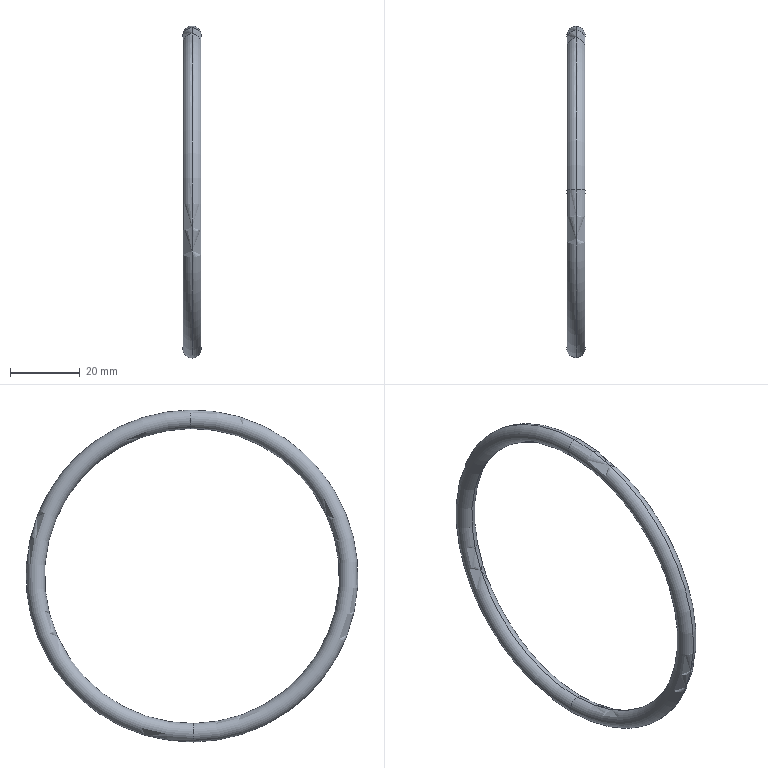Component | SolidWorks | SpringClipRubberRing-1 | 1 solid | 4 faces | box 5.3 x 95.03 x 95.03 mm | volume 6219 mm3 | torus 4 | material Silicone Rubber
STEP:
#1=COLOUR_RGB('',0.7922,0.8196,0.9333);
#2=FILL_AREA_STYLE_COLOUR('',#1);
#3=FILL_AREA_STYLE('',(#2));
#4=SURFACE_STYLE_FILL_AREA(#3);
#5=SURFACE_SIDE_STYLE('',(#4));
#6=SURFACE_STYLE_USAGE(.BOTH.,#5);
#7=PRESENTATION_STYLE_ASSIGNMENT((#6));
#8=CARTESIAN_POINT('',(19.367,-0.02012,-1.871));
#9=VERTEX_POINT('',#8);
#10=CARTESIAN_POINT('',(19.367,-0.01787,-1.662));
#11=VERTEX_POINT('',#10);
#12=CARTESIAN_POINT('',(19.367,-0.01899,-1.766));
#13=DIRECTION('',(0.,0.9999,-0.01075));
#14=DIRECTION('',(0.,0.01075,0.9999));
#15=AXIS2_PLACEMENT_3D('',#12,#13,#14);
#16=CIRCLE('',#15,0.1043);
#17=EDGE_CURVE('',#9,#11,#16,.T.);
#18=ORIENTED_EDGE('',*,*,#17,.F.);
#19=CARTESIAN_POINT('',(19.367,0.02012,1.871));
#20=VERTEX_POINT('',#19);
#21=CARTESIAN_POINT('',(19.367,0.,-0.));
#22=DIRECTION('',(-1.,0.,0.));
#23=DIRECTION('',(0.,0.,1.));
#24=AXIS2_PLACEMENT_3D('',#21,#22,#23);
#25=CIRCLE('',#24,1.871);
#26=EDGE_CURVE('',#9,#20,#25,.T.);
#27=ORIENTED_EDGE('',*,*,#26,.T.);
#28=CARTESIAN_POINT('',(19.367,0.01787,1.662));
#29=VERTEX_POINT('',#28);
#30=CARTESIAN_POINT('',(19.367,0.01899,1.766));
#31=DIRECTION('',(0.,-0.9999,0.01075));
#32=DIRECTION('',(0.,-0.01075,-0.9999));
#33=AXIS2_PLACEMENT_3D('',#30,#31,#32);
#34=CIRCLE('',#33,0.1043);
#35=EDGE_CURVE('',#20,#29,#34,.T.);
#36=ORIENTED_EDGE('',*,*,#35,.T.);
#37=CARTESIAN_POINT('',(19.367,0.,-0.));
#38=DIRECTION('',(-1.,0.,0.));
#39=DIRECTION('',(0.,0.,1.));
#40=AXIS2_PLACEMENT_3D('',#37,#38,#39);
#41=CIRCLE('',#40,1.662);
#42=EDGE_CURVE('',#11,#29,#41,.T.);
#43=ORIENTED_EDGE('',*,*,#42,.F.);
#44=EDGE_LOOP('',(#18,#27,#36,#43));
#45=FACE_OUTER_BOUND('',#44,.T.);
#46=CARTESIAN_POINT('',(19.367,0.,-0.));
#47=DIRECTION('',(-1.,0.,0.));
#48=DIRECTION('',(0.,0.01075,0.9999));
#49=AXIS2_PLACEMENT_3D('',#46,#47,#48);
#50=TOROIDAL_SURFACE('',#49,1.766,0.1043);
#51=ADVANCED_FACE('',(#45),#50,.T.);
#52=ORIENTED_EDGE('',*,*,#35,.F.);
#53=CARTESIAN_POINT('',(19.367,0.,-0.));
#54=DIRECTION('',(-1.,0.,0.));
#55=DIRECTION('',(0.,0.,1.));
#56=AXIS2_PLACEMENT_3D('',#53,#54,#55);
#57=CIRCLE('',#56,1.871);
#58=EDGE_CURVE('',#20,#9,#57,.T.);
#59=ORIENTED_EDGE('',*,*,#58,.T.);
#60=ORIENTED_EDGE('',*,*,#17,.T.);
#61=CARTESIAN_POINT('',(19.367,0.,-0.));
#62=DIRECTION('',(-1.,0.,0.));
#63=DIRECTION('',(0.,0.,1.));
#64=AXIS2_PLACEMENT_3D('',#61,#62,#63);
#65=CIRCLE('',#64,1.662);
#66=EDGE_CURVE('',#29,#11,#65,.T.);
#67=ORIENTED_EDGE('',*,*,#66,.F.);
#68=EDGE_LOOP('',(#52,#59,#60,#67));
#69=FACE_OUTER_BOUND('',#68,.T.);
#70=CARTESIAN_POINT('',(19.367,0.,-0.));
#71=DIRECTION('',(-1.,0.,0.));
#72=DIRECTION('',(0.,0.01075,0.9999));
#73=AXIS2_PLACEMENT_3D('',#70,#71,#72);
#74=TOROIDAL_SURFACE('',#73,1.766,0.1043);
#75=ADVANCED_FACE('',(#69),#74,.T.);
#76=ORIENTED_EDGE('',*,*,#58,.F.);
#77=CARTESIAN_POINT('',(19.367,0.01899,1.766));
#78=DIRECTION('',(0.,-0.9999,0.01075));
#79=DIRECTION('',(0.,-0.01075,-0.9999));
#80=AXIS2_PLACEMENT_3D('',#77,#78,#79);
#81=CIRCLE('',#80,0.1043);
#82=EDGE_CURVE('',#29,#20,#81,.T.);
#83=ORIENTED_EDGE('',*,*,#82,.F.);
#84=ORIENTED_EDGE('',*,*,#66,.T.);
#85=CARTESIAN_POINT('',(19.367,-0.01899,-1.766));
#86=DIRECTION('',(0.,0.9999,-0.01075));
#87=DIRECTION('',(0.,0.01075,0.9999));
#88=AXIS2_PLACEMENT_3D('',#85,#86,#87);
#89=CIRCLE('',#88,0.1043);
#90=EDGE_CURVE('',#11,#9,#89,.T.);
#91=ORIENTED_EDGE('',*,*,#90,.T.);
#92=EDGE_LOOP('',(#76,#83,#84,#91));
#93=FACE_OUTER_BOUND('',#92,.T.);
#94=CARTESIAN_POINT('',(19.367,0.,-0.));
#95=DIRECTION('',(-1.,0.,0.));
#96=DIRECTION('',(0.,0.01075,0.9999));
#97=AXIS2_PLACEMENT_3D('',#94,#95,#96);
#98=TOROIDAL_SURFACE('',#97,1.766,0.1043);
#99=ADVANCED_FACE('',(#93),#98,.T.);
#100=ORIENTED_EDGE('',*,*,#26,.F.);
#101=ORIENTED_EDGE('',*,*,#90,.F.);
#102=ORIENTED_EDGE('',*,*,#42,.T.);
#103=ORIENTED_EDGE('',*,*,#82,.T.);
#104=EDGE_LOOP('',(#100,#101,#102,#103));
#105=FACE_OUTER_BOUND('',#104,.T.);
#106=CARTESIAN_POINT('',(19.367,0.,-0.));
#107=DIRECTION('',(-1.,0.,0.));
#108=DIRECTION('',(0.,0.01075,0.9999));
#109=AXIS2_PLACEMENT_3D('',#106,#107,#108);
#110=TOROIDAL_SURFACE('',#109,1.766,0.1043);
#111=ADVANCED_FACE('',(#105),#110,.T.);
#112=CLOSED_SHELL('',(#51,#75,#99,#111));
#113=MANIFOLD_SOLID_BREP('',#112);
#114=STYLED_ITEM('',(#7),#113);
#115=PRESENTATION_LAYER_ASSIGNMENT('','',(#114));
#116=CARTESIAN_POINT('',(0.,0.,0.));
#117=DIRECTION('',(0.,0.,1.));
#118=DIRECTION('',(1.,0.,0.));
#119=AXIS2_PLACEMENT_3D('',#116,#117,#118);
#120=(LENGTH_UNIT()NAMED_UNIT(*)SI_UNIT($,.METRE.));
#121=LENGTH_MEASURE_WITH_UNIT(LENGTH_MEASURE(0.0254),#120);
#122=DIMENSIONAL_EXPONENTS(1.,0.,0.,0.,0.,0.,0.);
#123=(CONVERSION_BASED_UNIT('',#121)LENGTH_UNIT()NAMED_UNIT(#122));
#124=UNCERTAINTY_MEASURE_WITH_UNIT(LENGTH_MEASURE(0.00001),#123,'','');
#125=(NAMED_UNIT(*)PLANE_ANGLE_UNIT()SI_UNIT($,.RADIAN.));
#126=(NAMED_UNIT(*)SI_UNIT($,.STERADIAN.)SOLID_ANGLE_UNIT());
#127=(GEOMETRIC_REPRESENTATION_CONTEXT(3)GLOBAL_UNCERTAINTY_ASSIGNED_CONTEXT((#124))GLOBAL_UNIT_ASSIGNED_CONTEXT((#123,#125,#126))REPRESENTATION_CONTEXT('',''));
#128=ADVANCED_BREP_SHAPE_REPRESENTATION('',(#113,#119),#127);
#129=(LENGTH_UNIT()NAMED_UNIT(*)SI_UNIT($,.METRE.));
#130=LENGTH_MEASURE_WITH_UNIT(LENGTH_MEASURE(0.0254),#129);
#131=DIMENSIONAL_EXPONENTS(1.,0.,0.,0.,0.,0.,0.);
#132=(CONVERSION_BASED_UNIT('',#130)LENGTH_UNIT()NAMED_UNIT(#131));
#133=UNCERTAINTY_MEASURE_WITH_UNIT(LENGTH_MEASURE(0.00001),#132,'','');
#134=(NAMED_UNIT(*)PLANE_ANGLE_UNIT()SI_UNIT($,.RADIAN.));
#135=(NAMED_UNIT(*)SI_UNIT($,.STERADIAN.)SOLID_ANGLE_UNIT());
#136=(GEOMETRIC_REPRESENTATION_CONTEXT(3)GLOBAL_UNCERTAINTY_ASSIGNED_CONTEXT((#133))GLOBAL_UNIT_ASSIGNED_CONTEXT((#132,#134,#135))REPRESENTATION_CONTEXT('',''));
#137=MECHANICAL_DESIGN_GEOMETRIC_PRESENTATION_REPRESENTATION('',(#114),#136);